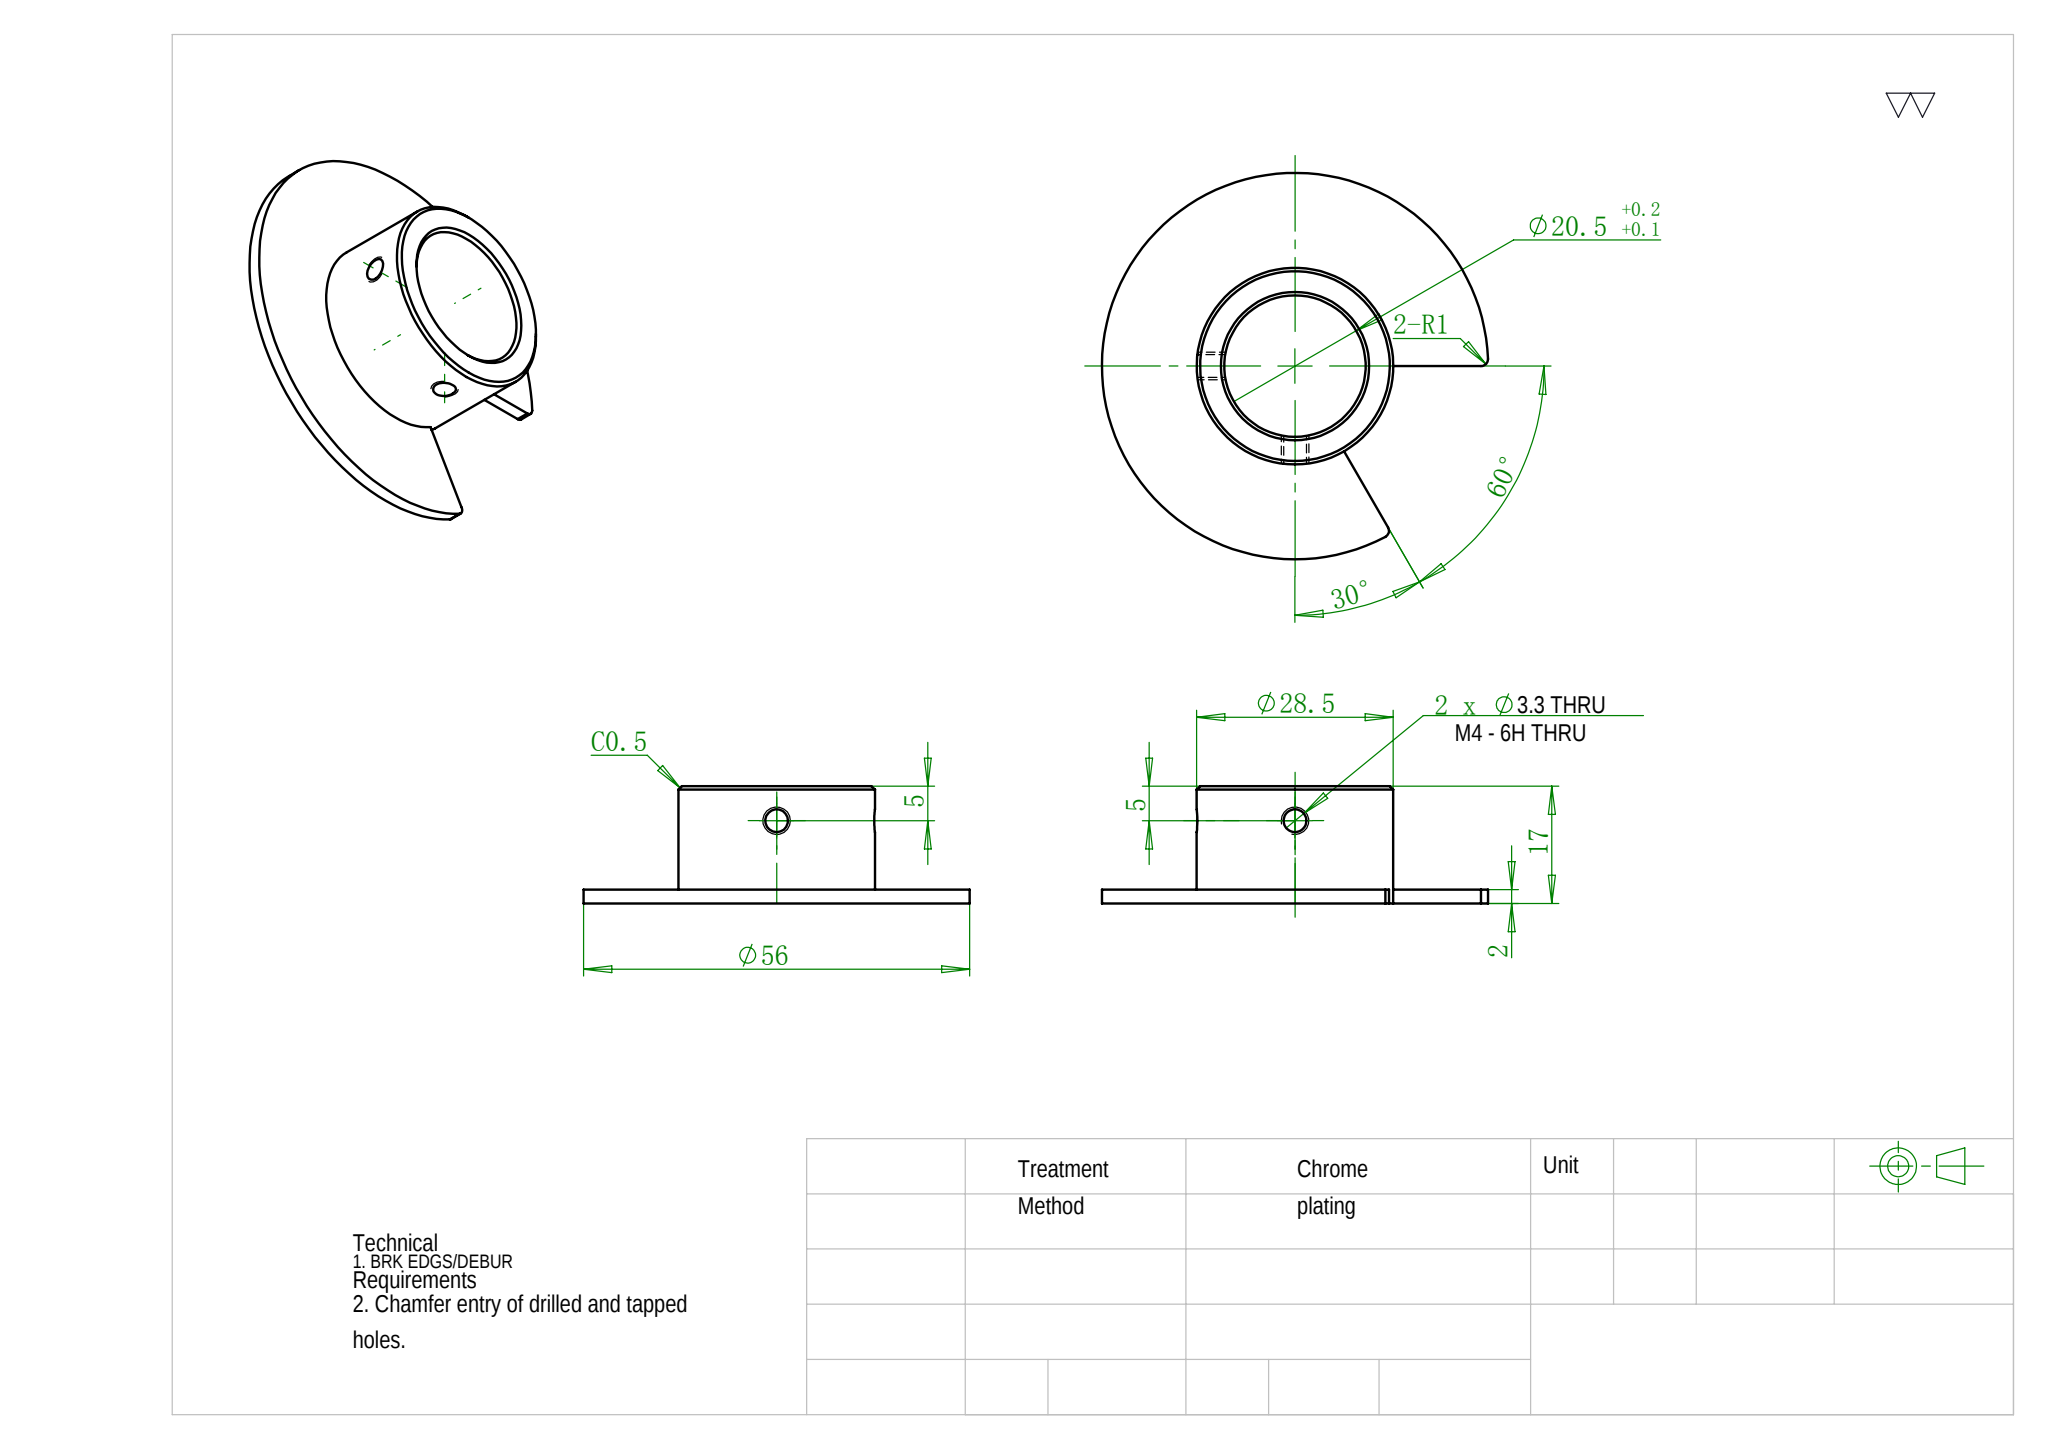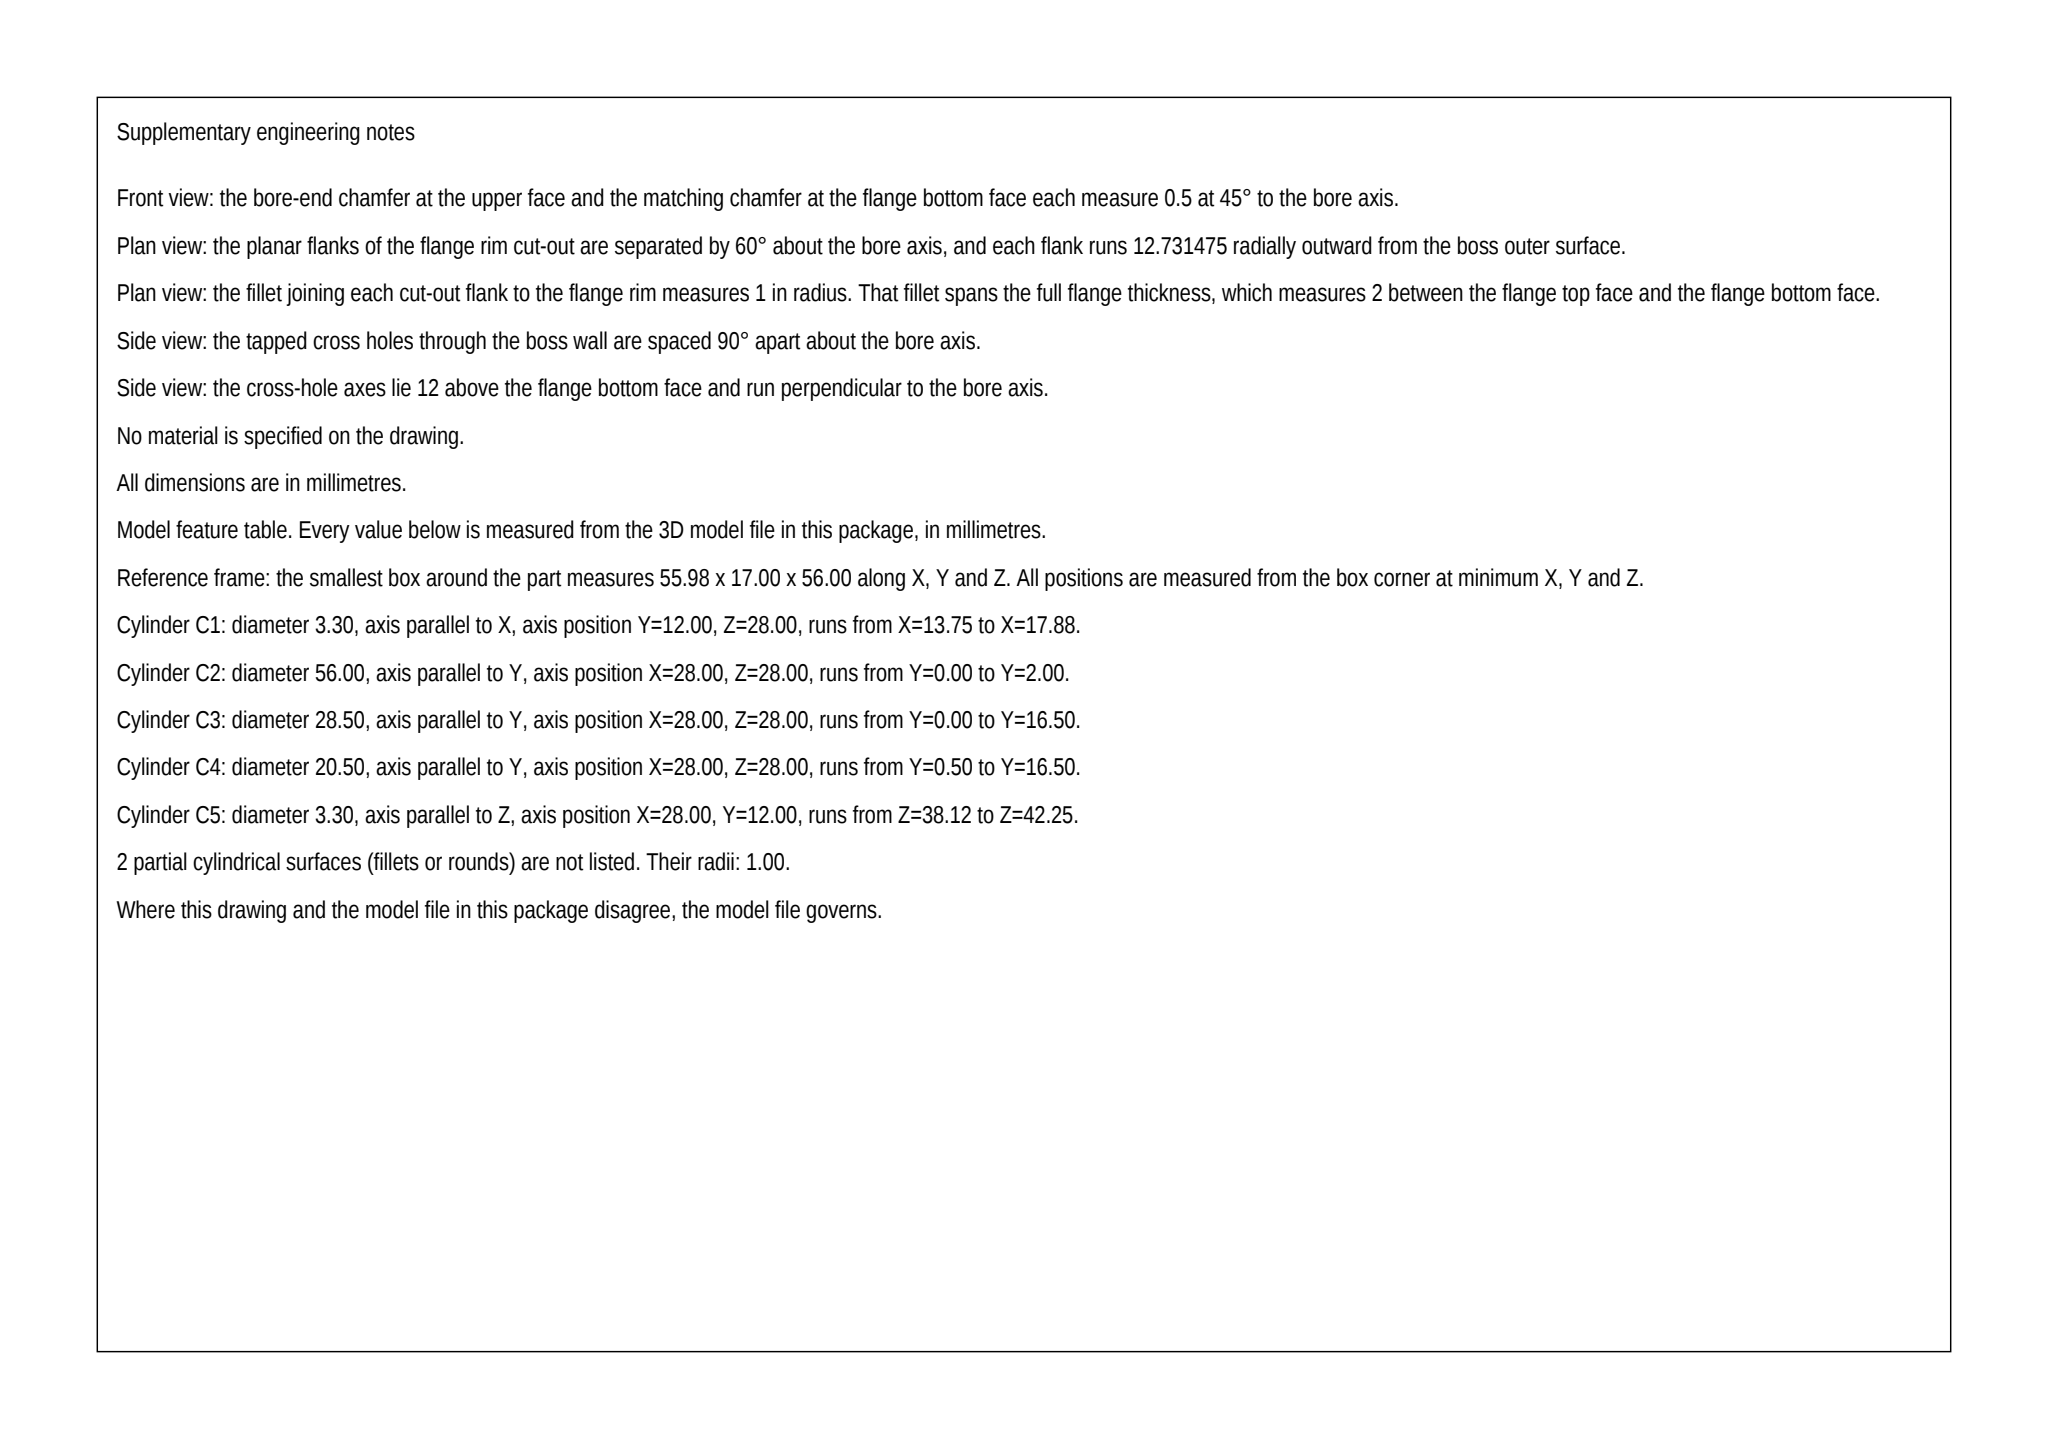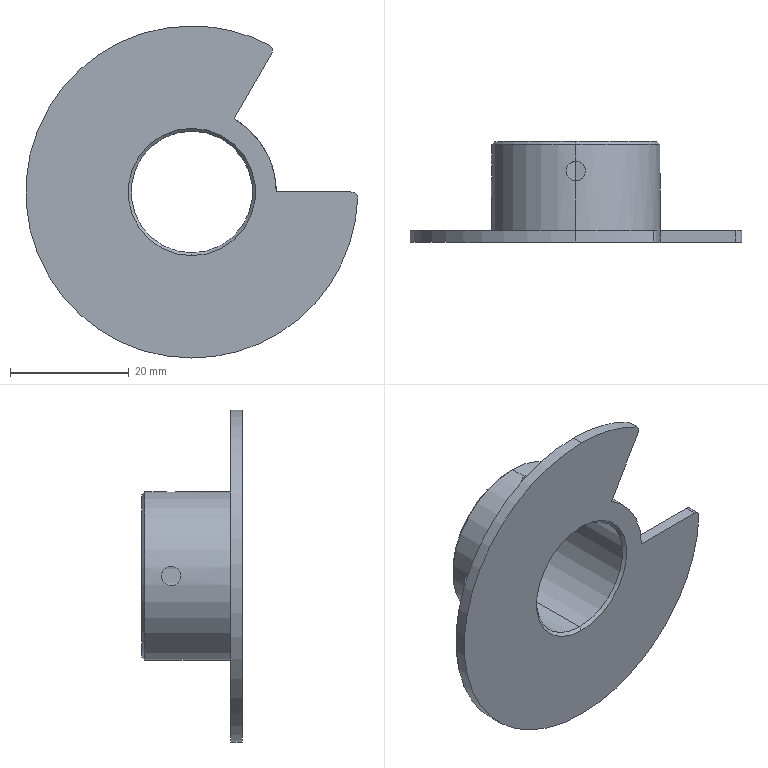Part | SolidWorks | mm | 1 solid | 24 faces | box 55.98 x 17 x 56 mm | volume 8179 mm3 | cylinder 13 | cone 6 | plane 5 | commonest cylinder face diameters 3.3 x4 56 x3 28.5 x2 20.5 x2 2 x2
build123d program:
from build123d import *

# Parameters (mm, degrees)
M4_TAPPED_HOLE1_REACH  = 60.112
M4_TAPPED_HOLE1_BORE_R = 1.65
CIRPATTERN1_COUNT      = 2
CIRPATTERN1_ANGLE      = 90
CHAMFER1_SIZE          = 0.5
CUT_EXTRUDE1_DEPTH     = 43.344
FILLET1_R              = 1


with BuildPart() as part:
    # Sketch1 → Revolve1 (revolve)
    with BuildSketch(Plane.XY, mode=Mode.PRIVATE) as revolve1_sk:
        Polygon((28, 0), (10.25, 0), (10.25, 17), (14.25, 17), (14.25, 2), (28, 2), align=None)
    revolve(revolve1_sk.sketch.rotate(Axis((0, 0, 0), (0, 1, 0)), 90), axis=Axis((0, 0, 0), (0, 1, 0)))

    # M4 Tapped Hole1 bore → M4 Tapped Hole1 (cut, up to next)
    with BuildSketch(Plane.XY.offset(20), mode=Mode.PRIVATE) as m4_tapped_hole1_sk1:
        with Locations((0, 12)):
            Circle(M4_TAPPED_HOLE1_BORE_R)
    m4_tapped_hole1_tool1 = extrude(m4_tapped_hole1_sk1.sketch, amount=-M4_TAPPED_HOLE1_REACH, mode=Mode.PRIVATE) & part.part
    m4_tapped_hole1 = m4_tapped_hole1_tool1.solids().sort_by_distance((0, 12, 20))[0]
    add(m4_tapped_hole1, mode=Mode.SUBTRACT)

    # CirPattern1: M4 Tapped Hole1 ×2 about axis
    cirpattern1_axis = Axis((0, 0, 0), (0, -1, 0))
    for i in range(1, CIRPATTERN1_COUNT):
        add(m4_tapped_hole1.rotate(cirpattern1_axis, i * CIRPATTERN1_ANGLE / (CIRPATTERN1_COUNT - 1)), mode=Mode.SUBTRACT)

    # Chamfer1
    chamfer1_edges = [part.edges().sort_by_distance(p)[0] for p in [
        (0, 0, 10.25),
        (0, 17, 14.25),
        (0, 17, 10.25),
    ]]
    chamfer(chamfer1_edges, length=CHAMFER1_SIZE)

    # Sketch4 → Cut-Extrude1 (cut, through all)
    with BuildSketch(Plane(origin=(0, 2, 0), x_dir=(1, 0, 0), z_dir=(0, 1, 0))):
        with BuildLine():
            Line((14.25, 0), (28, 0))
            ThreePointArc((28, 0), (24.249, -14), (14, -24.249))
            Line((14, -24.249), (7.125, -12.341))
            ThreePointArc((7.125, -12.341), (12.341, -7.125), (14.25, 0))
        make_face()
    extrude(amount=-CUT_EXTRUDE1_DEPTH, mode=Mode.SUBTRACT)

    # Fillet1
    fillet1_edges = [part.edges().sort_by_distance(p)[0] for p in [
        (28, 1, 0),
        (14, 1, 24.249),
    ]]
    fillet(fillet1_edges, radius=FILLET1_R)


solid = part.part